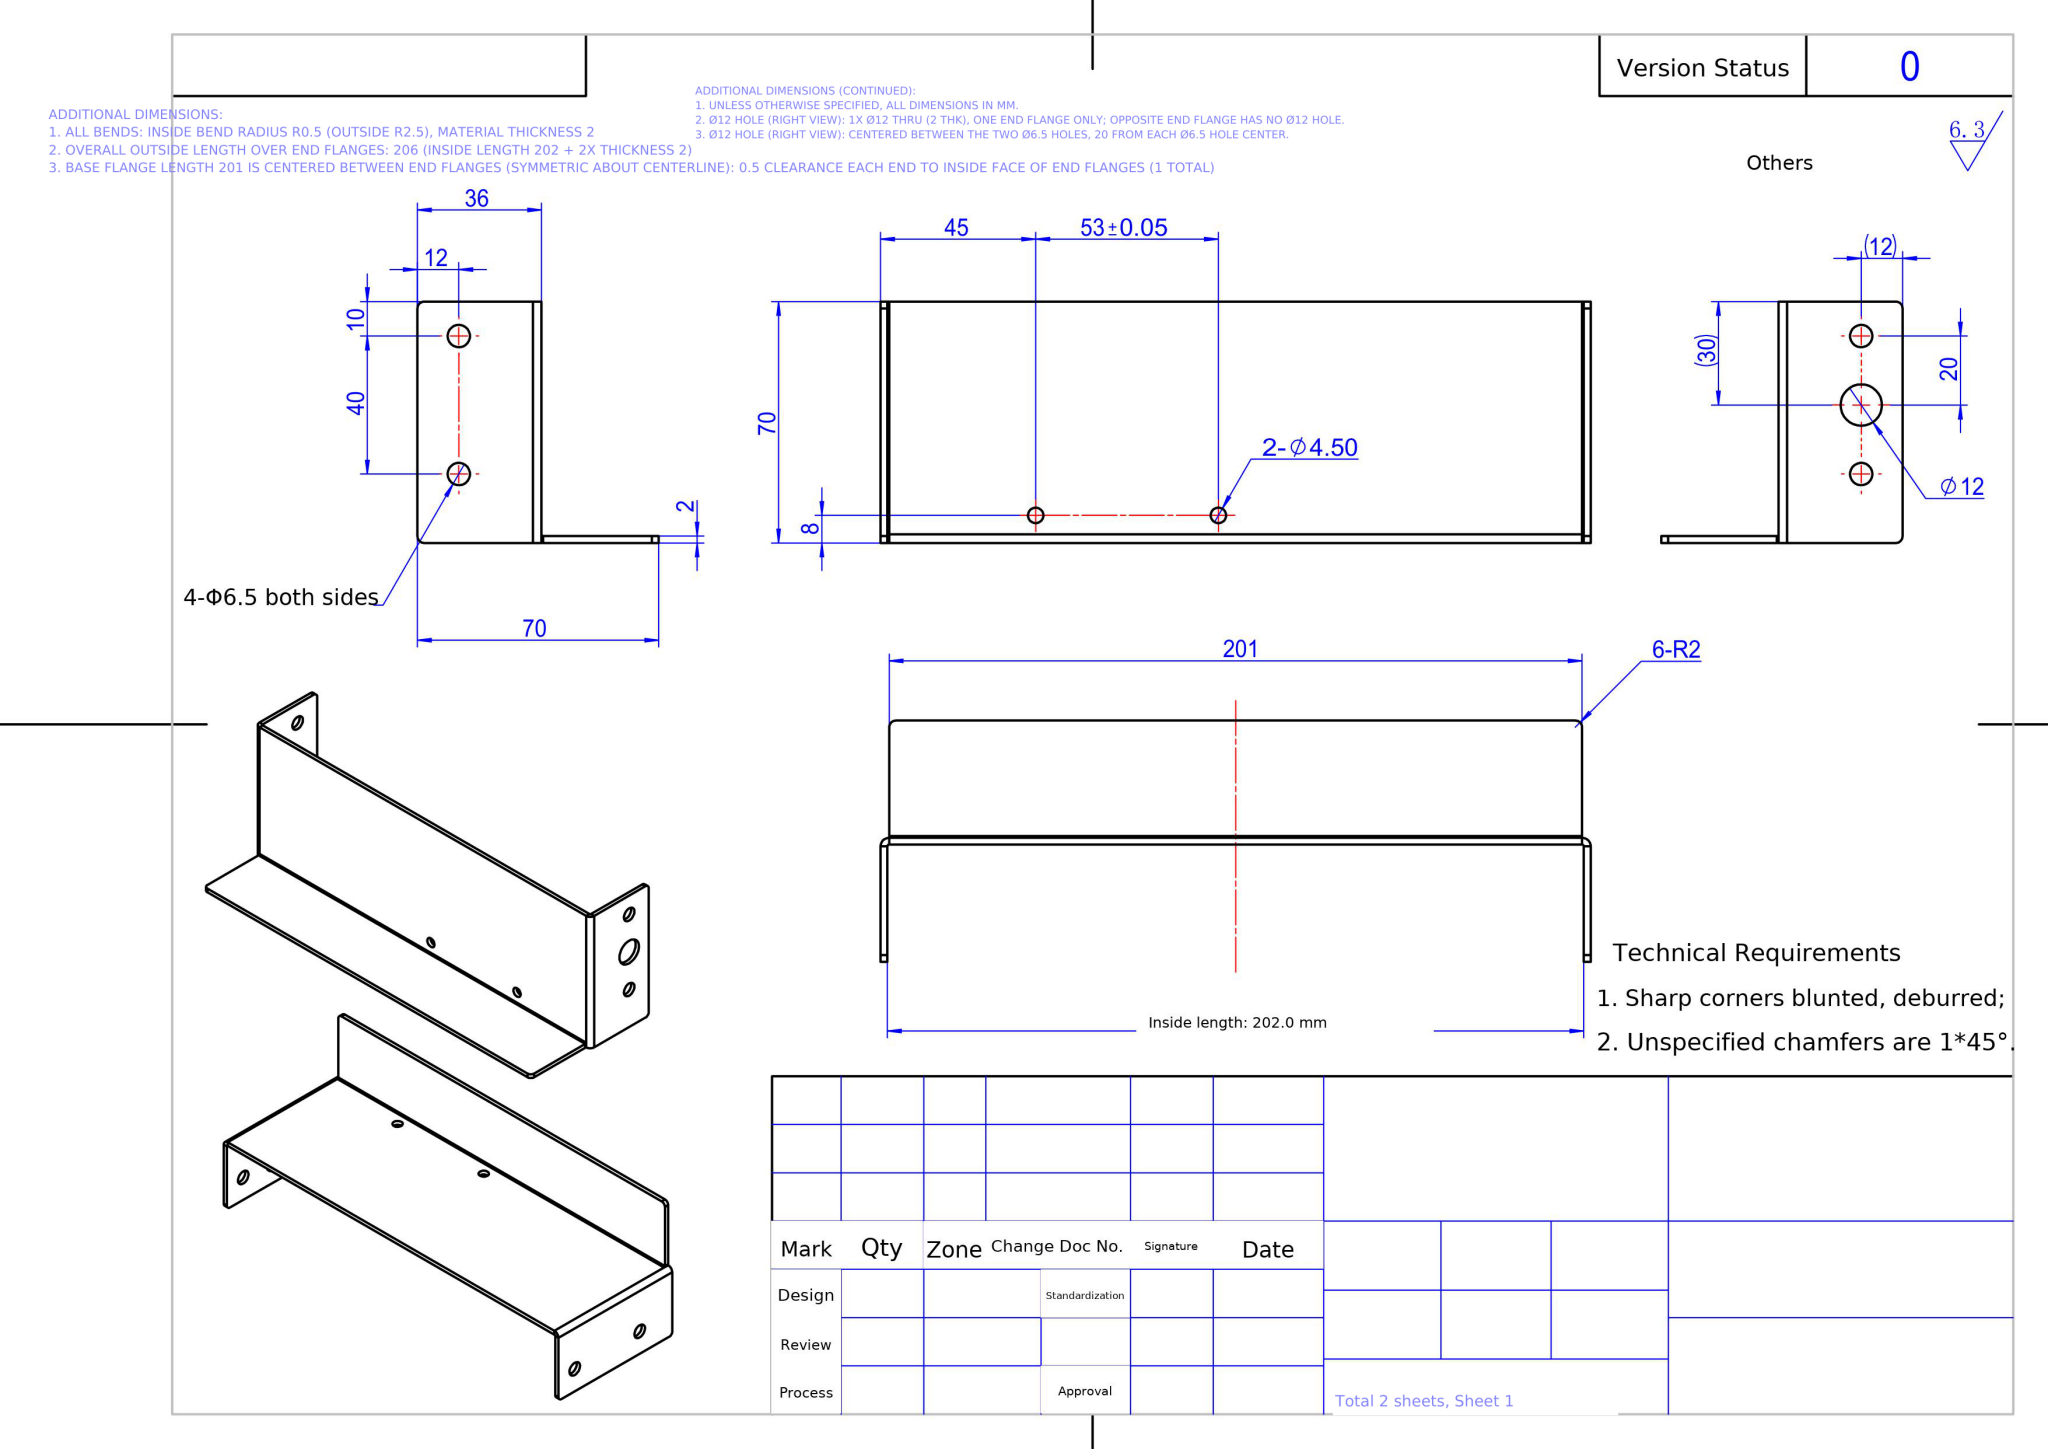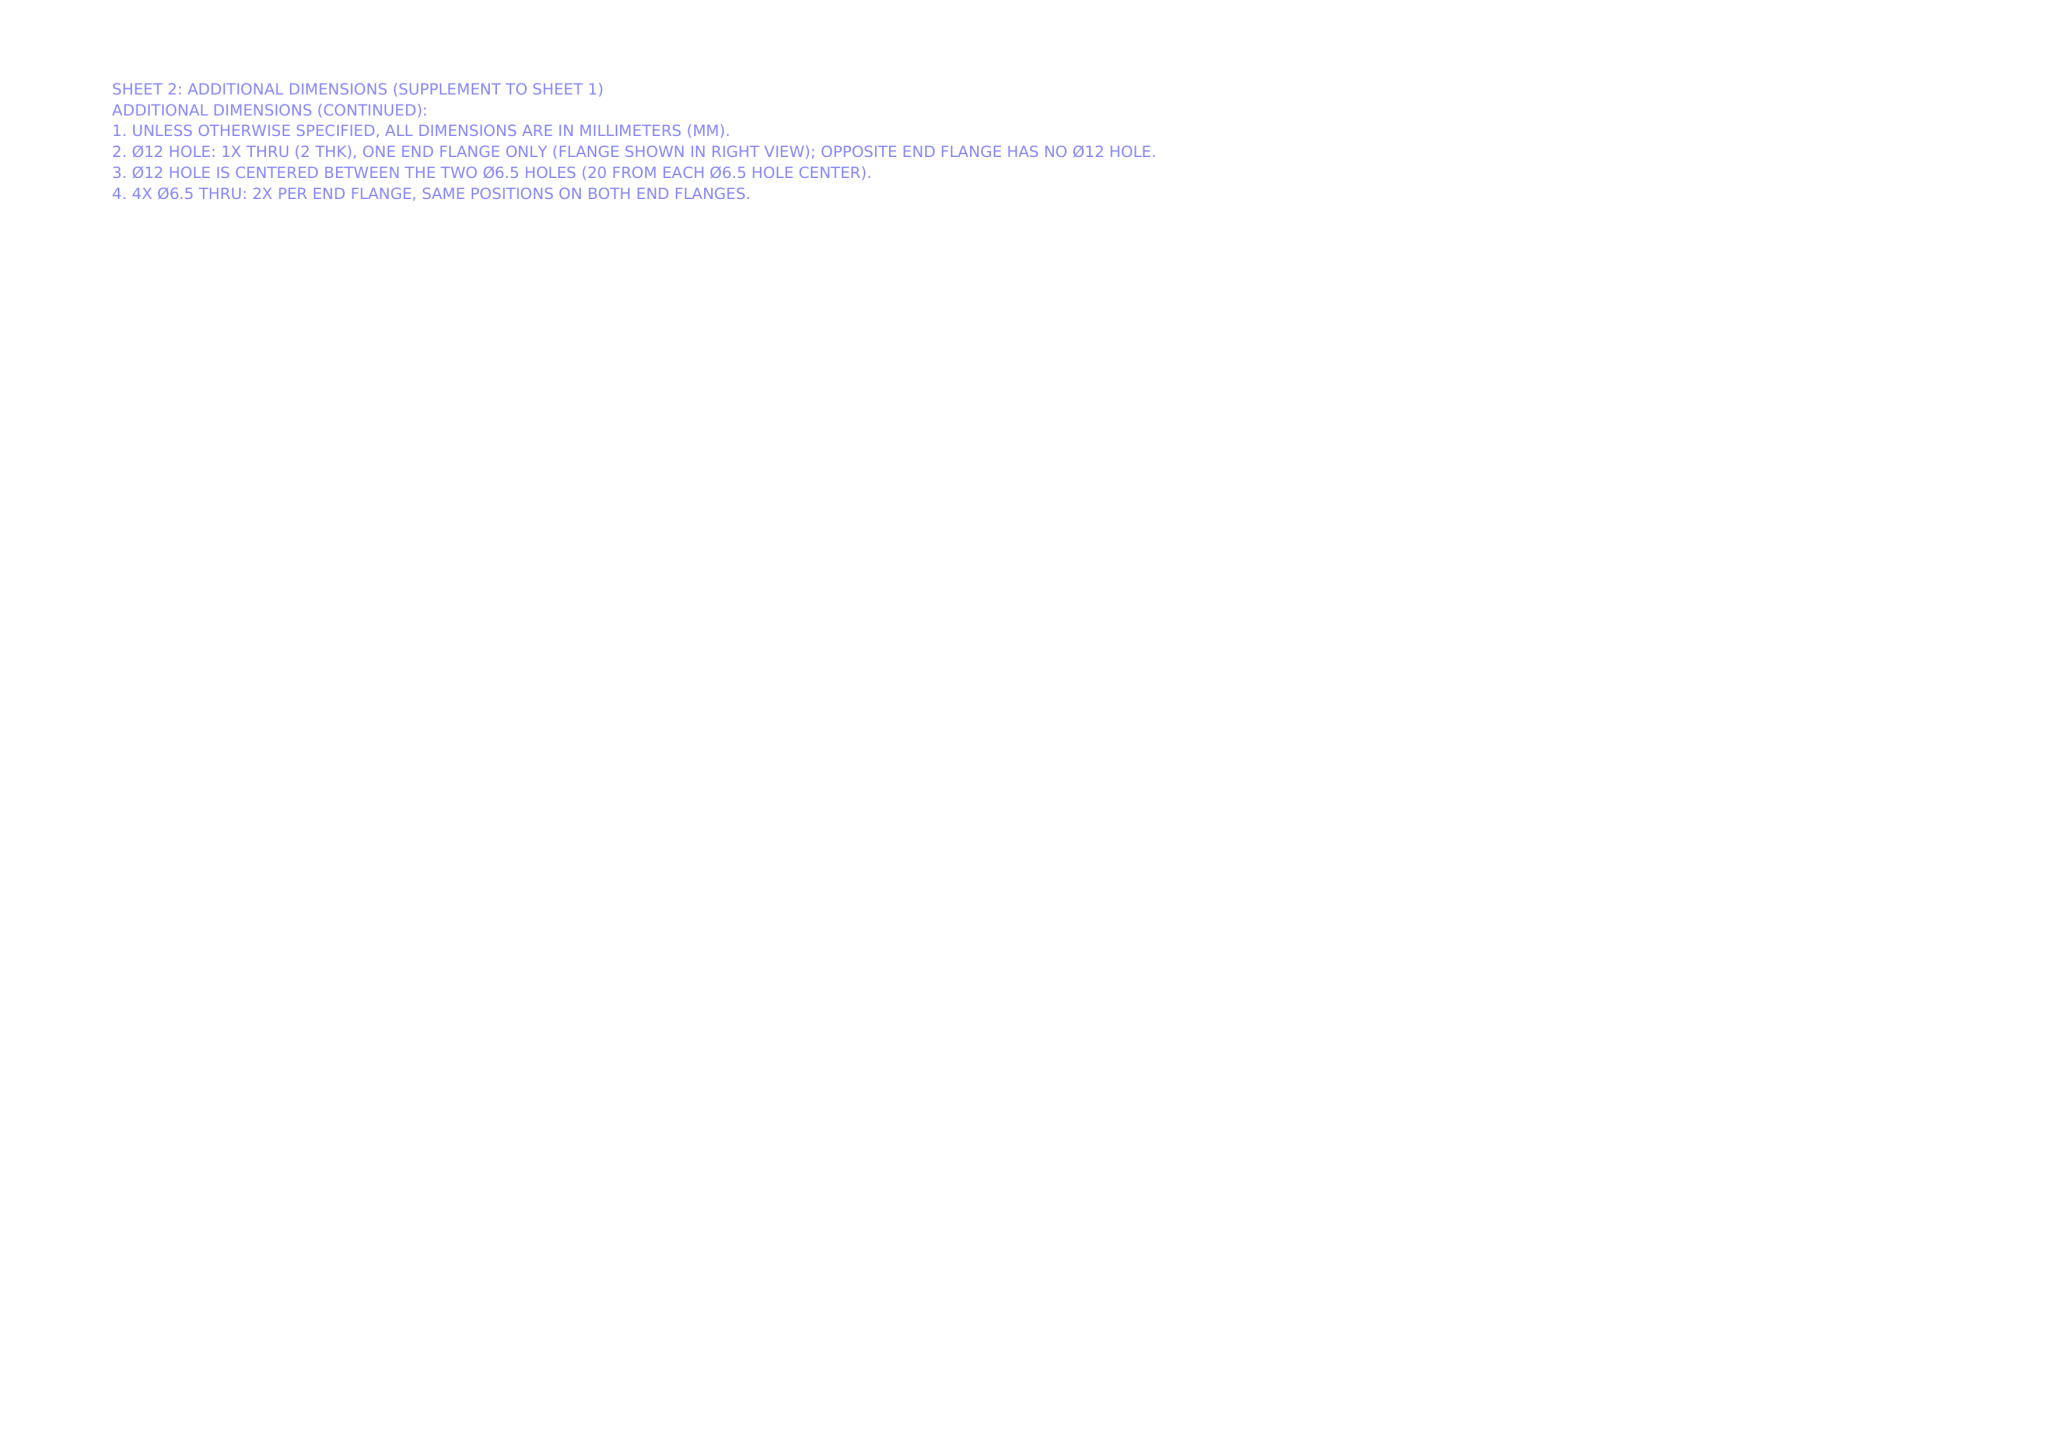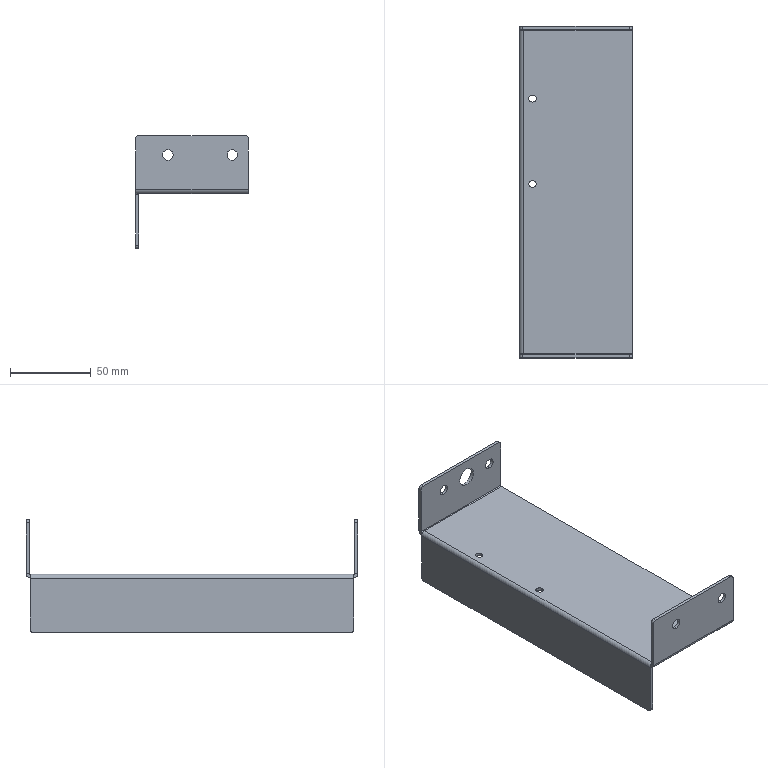Part | NX | mm | 1 solid | 52 faces | box 70 x 206 x 70 mm | volume 51023 mm3 | cylinder 26 | plane 26 | commonest cylinder face diameters 6.5 x8 4 x6 4.5 x4 5 x3 1 x3 12 x2